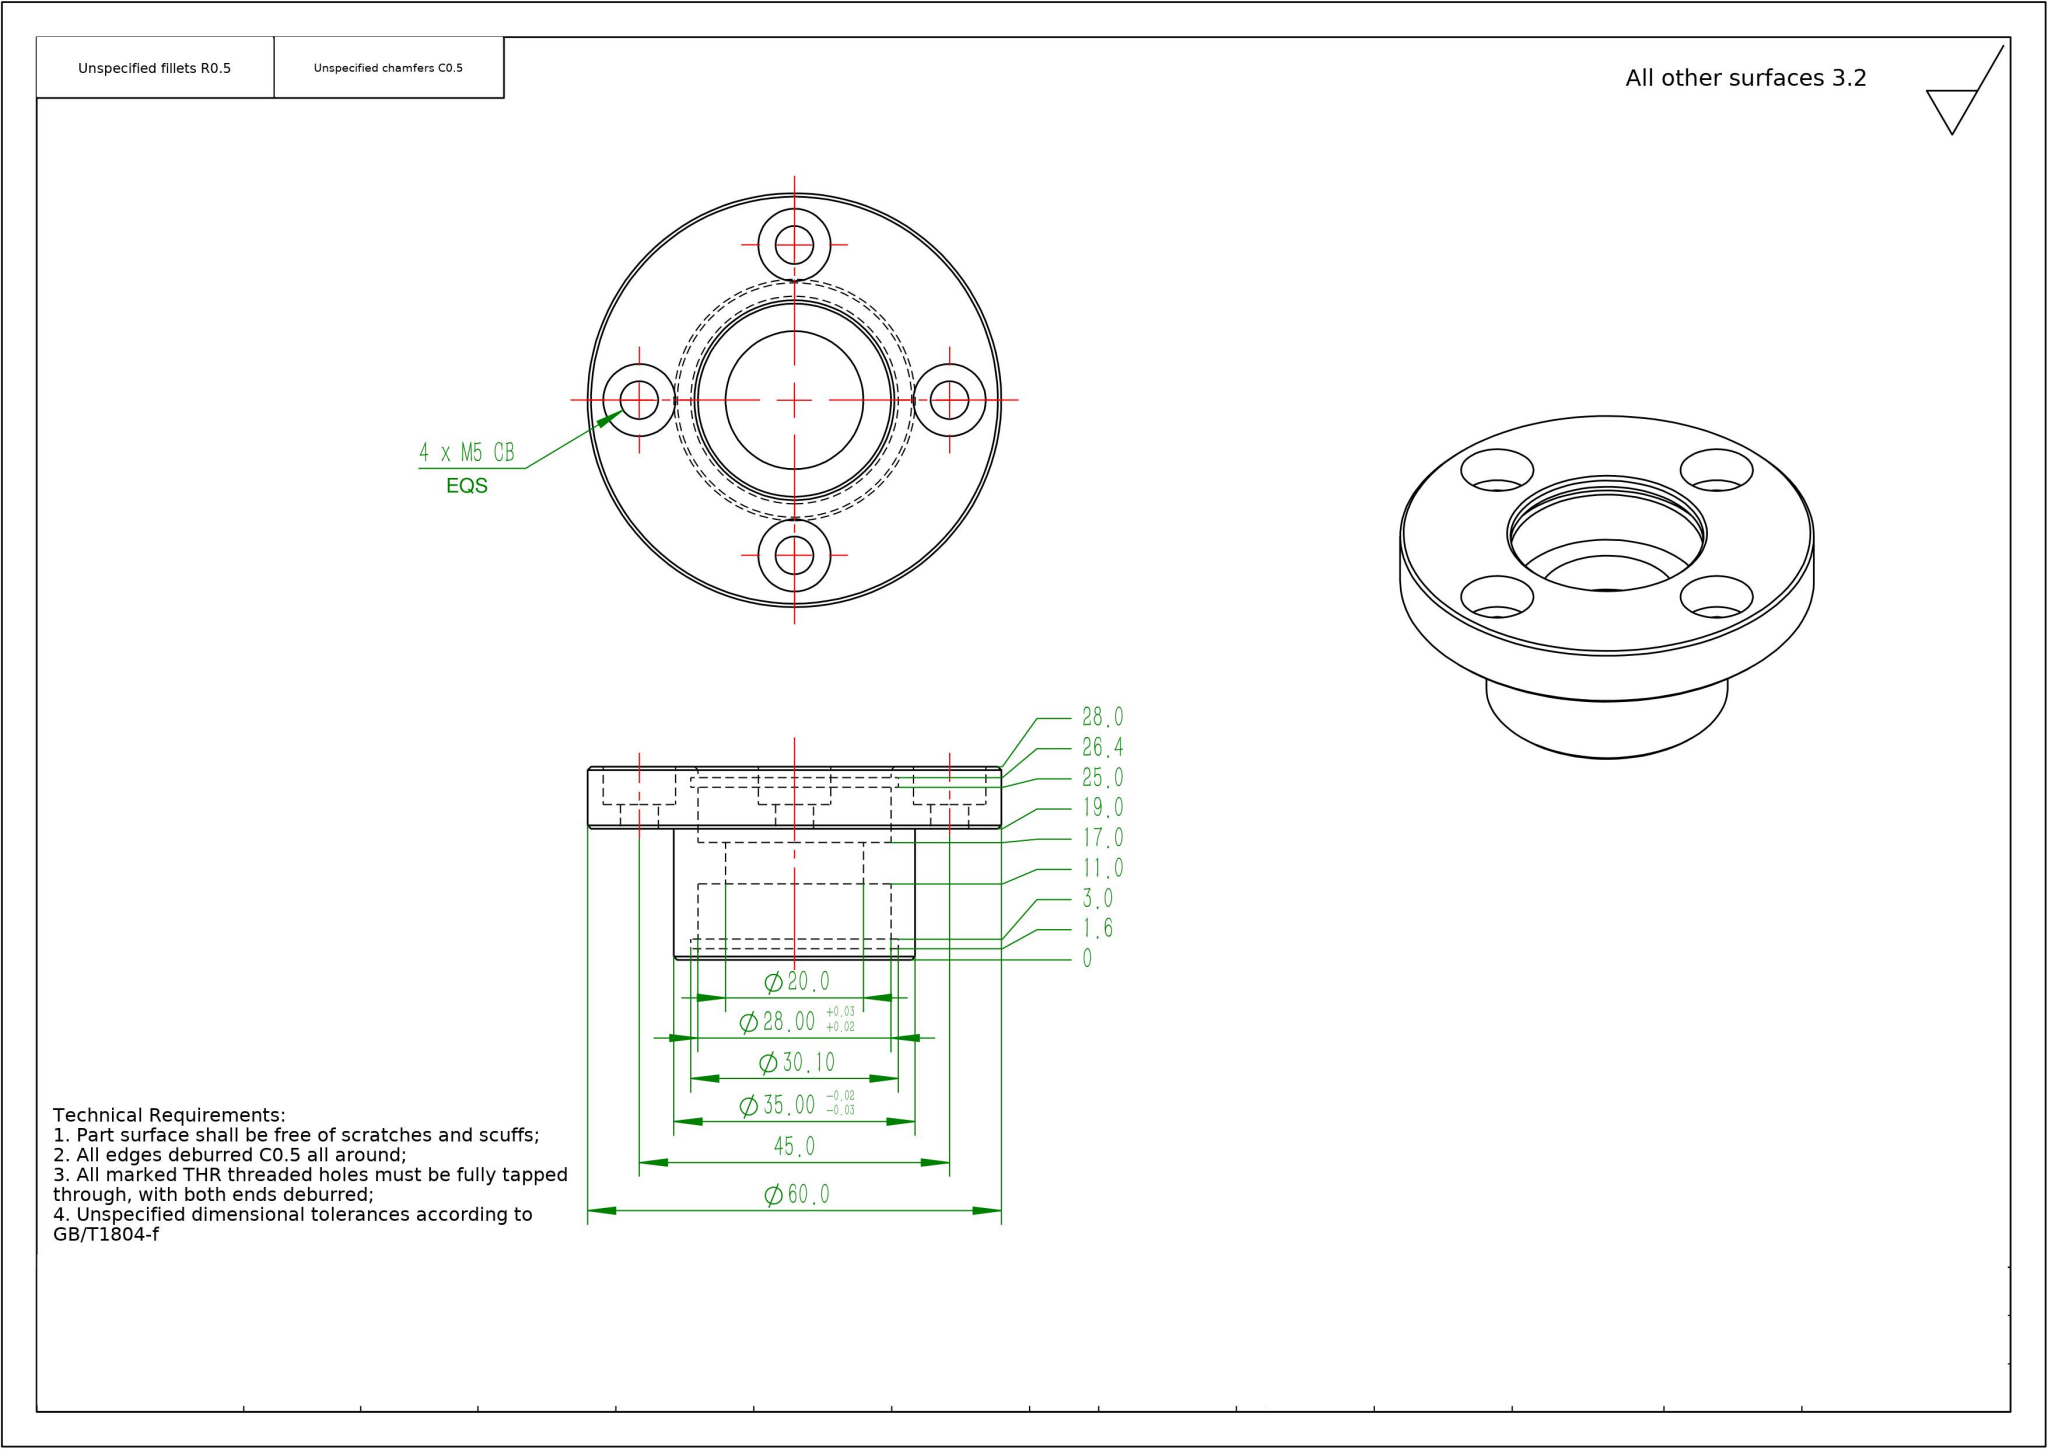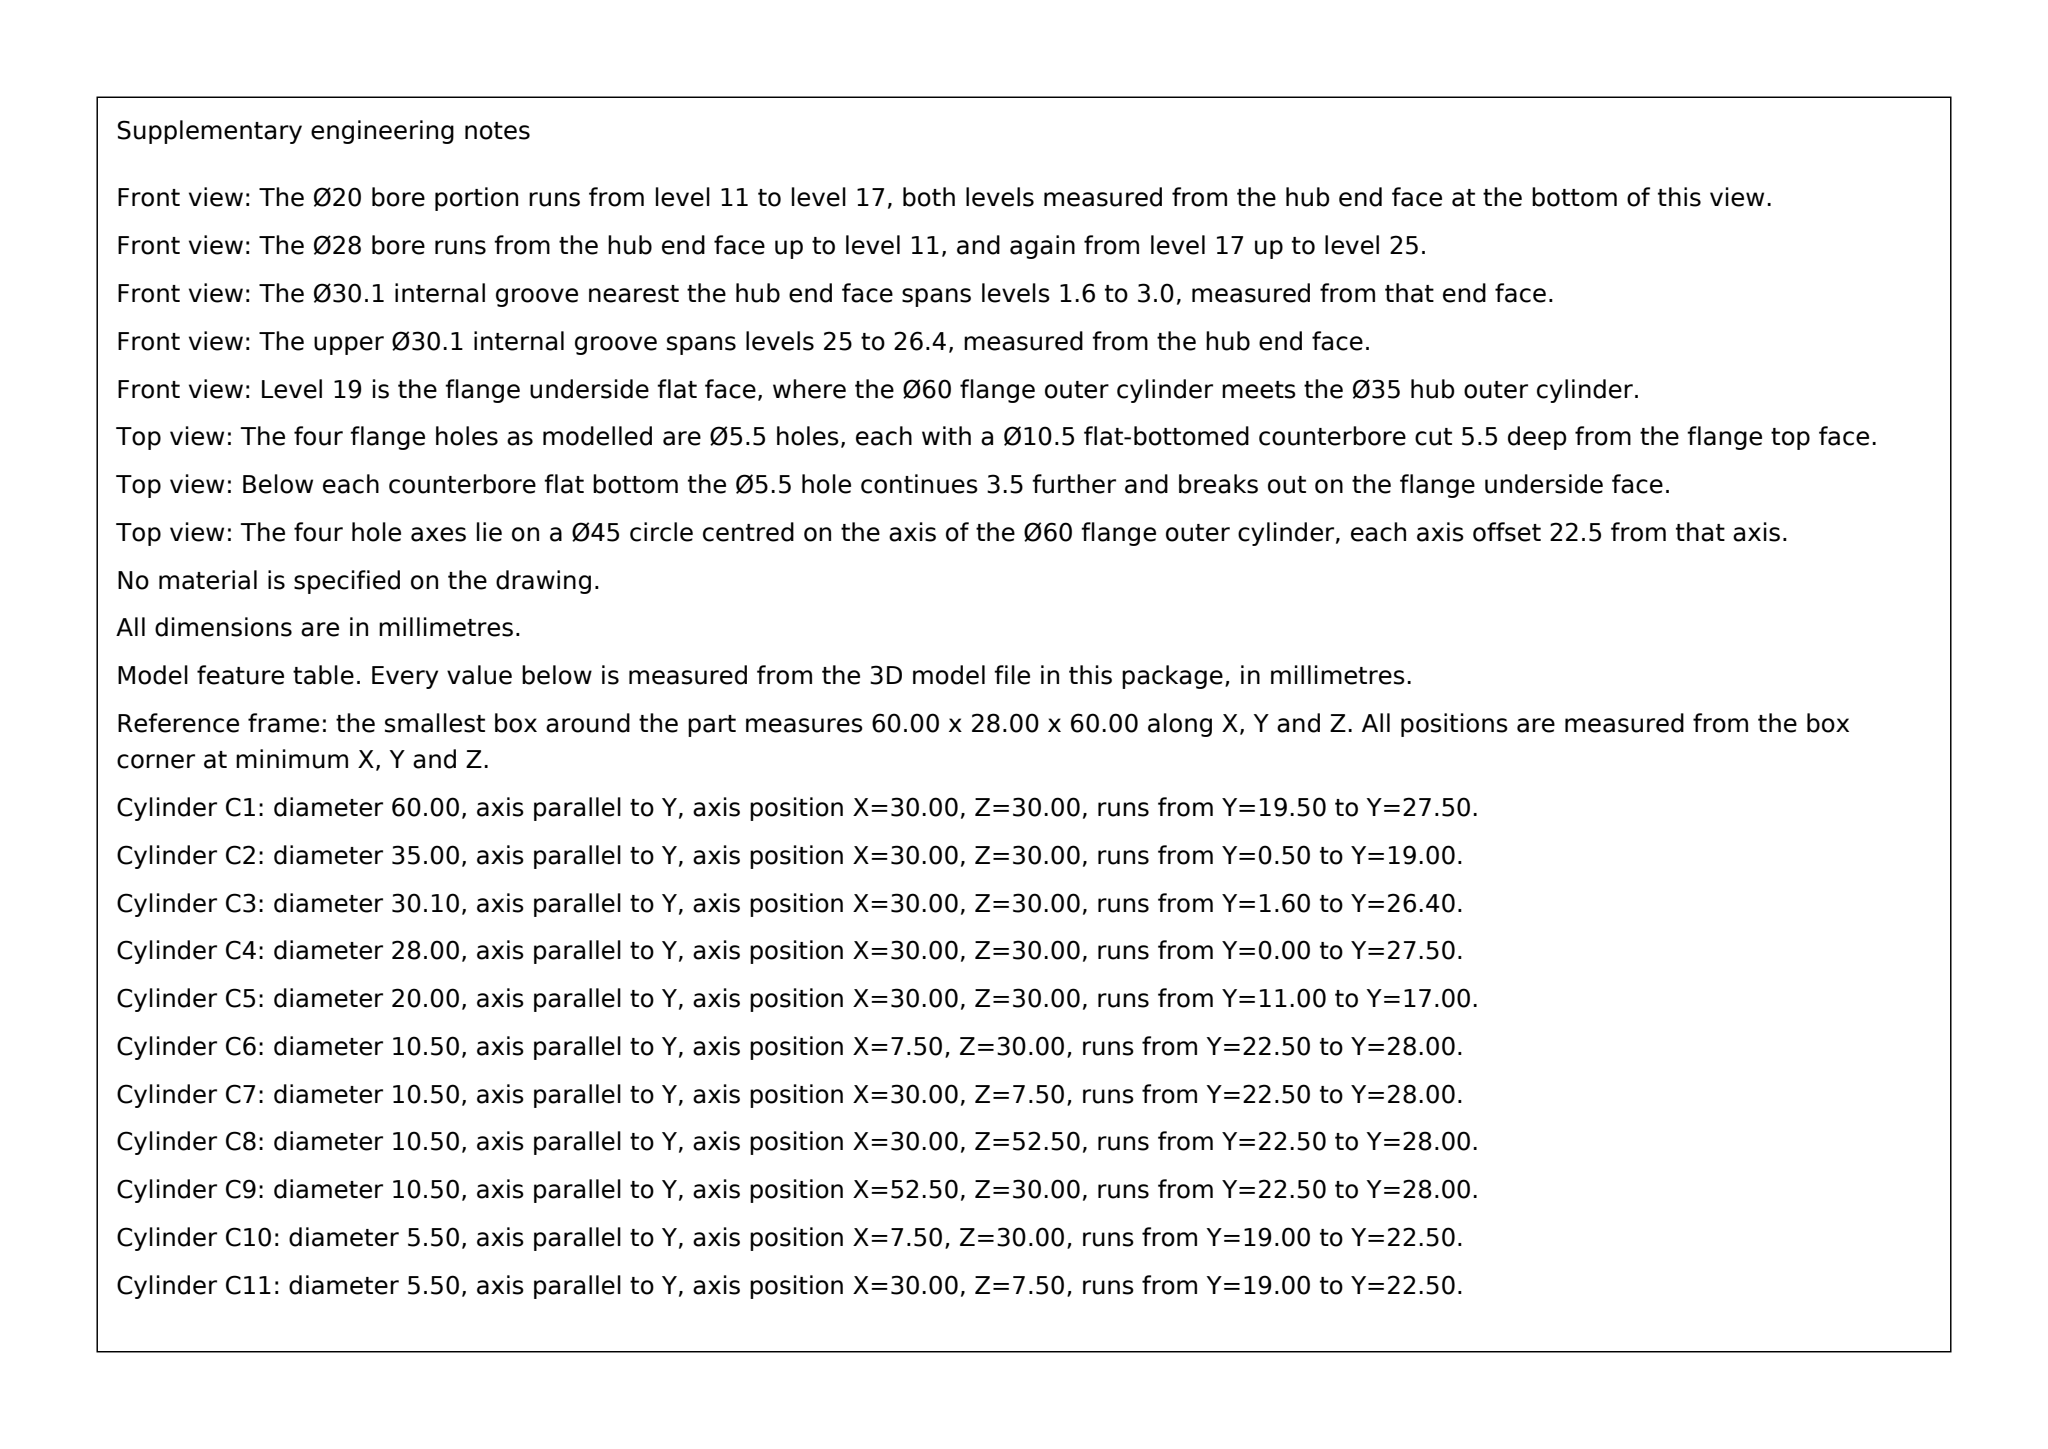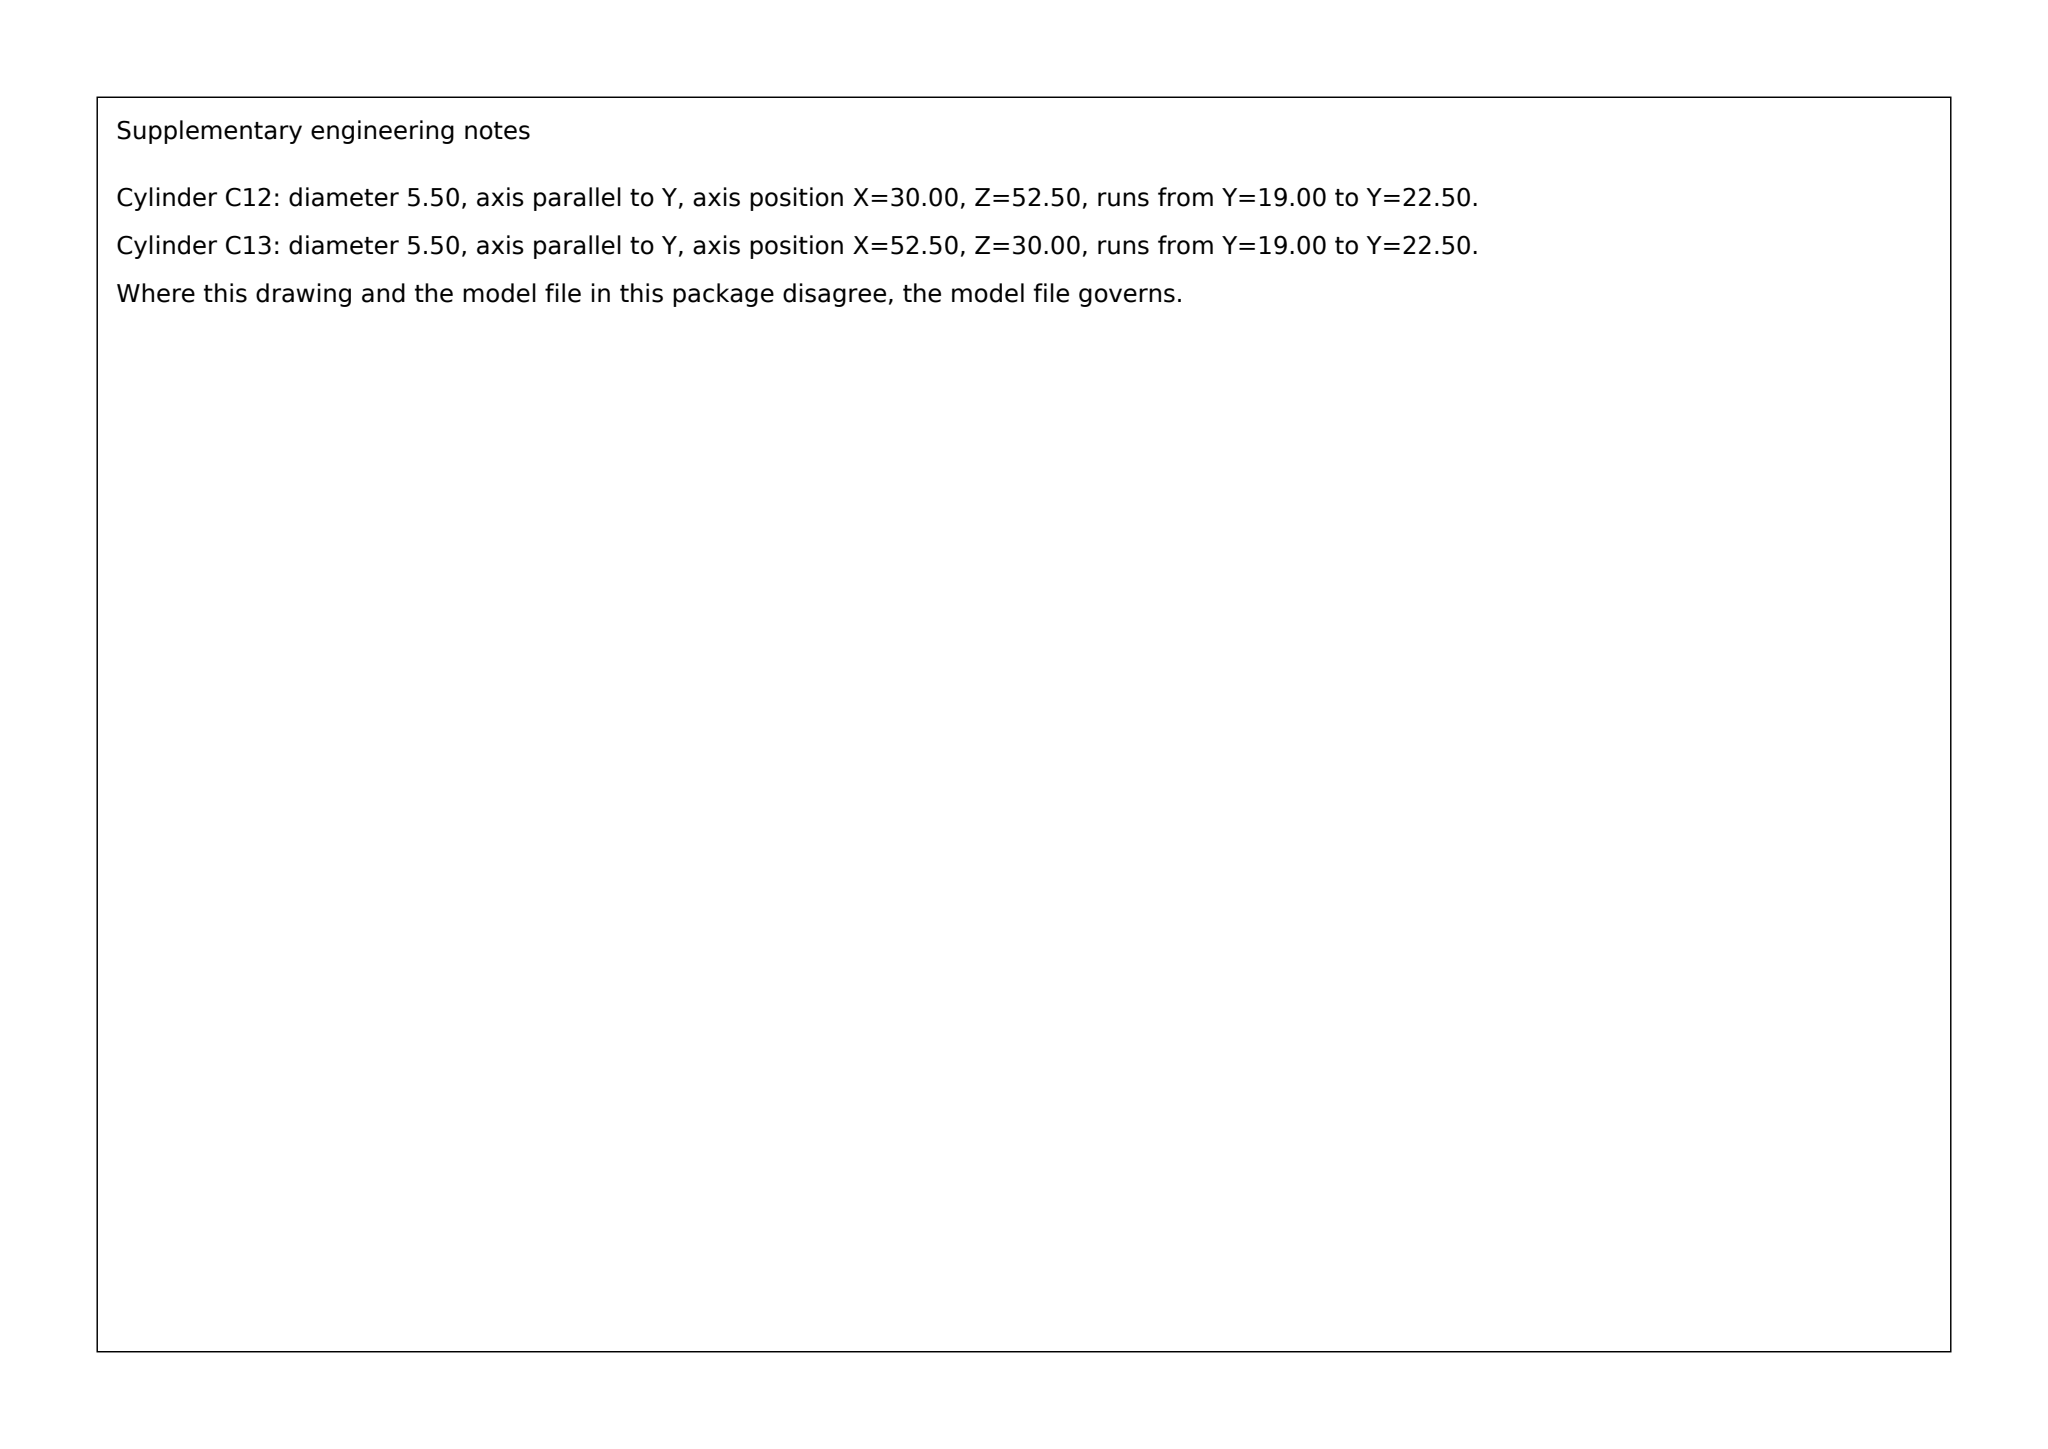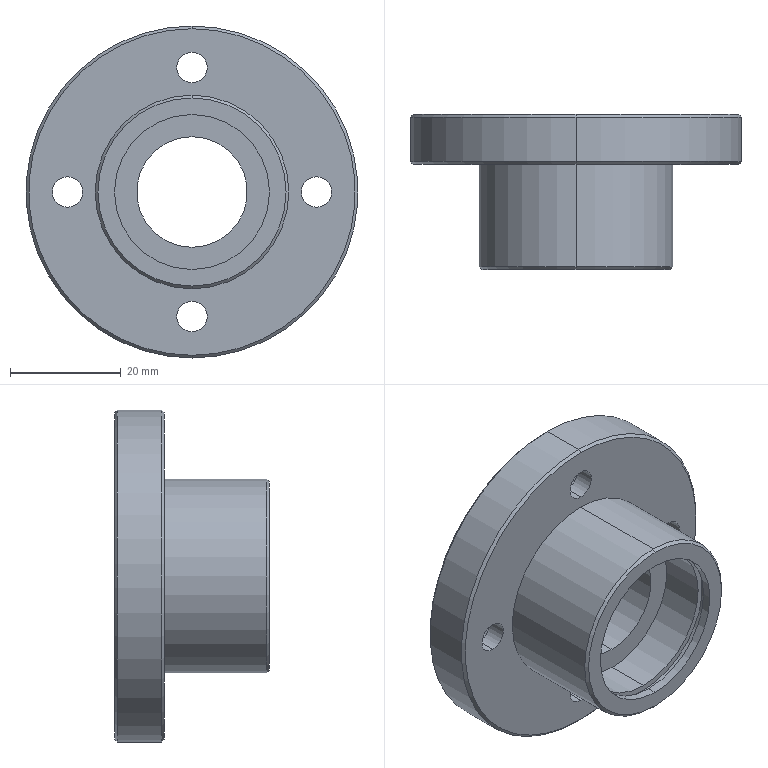Part | SolidWorks | mm | 1 solid | 55 faces | box 60 x 28 x 60 mm | volume 25718 mm3 | cylinder 34 | plane 13 | cone 8 | commonest cylinder face diameters 10.5 x8 28 x8 5.5 x8 30.1 x4 60 x2 20 x2 35 x2
Drawing notes:
4X C'BORE Ø10.5, EQ SP ON Ø45 B.C. | from the solid: cyl dia 10.5 axis y at (7.5,30),(30,7.5),(30,52.5),(52.5,30); R22.5 from axis (30,30) = Ø45 BC
4X C'BORE Ø10.5 DP 5.5 FROM 28.0 TOP FACE; FLOOR AT 22.5 | from the solid: cyl dia 10.5 len 5.5; planes y=28.0 (top) and y=22.5 (4X cbore floors)
4X Ø5.5 THRU TO C'BORE (22.5 TO 19.0 FLANGE UNDERSIDE) | from the solid: cyl dia 5.5 axis y len 3.5, between planes y=22.5 and y=19.0
INT THR MAJOR Ø30.10, THD LG 8.0 (17.0 TO 25.0 LEVELS) | from the solid: dia 30.10 thread-relief cyls (4) interleaved with dia 28.00 cyls len 8.0 between planes y=17.0 and y=25.0
INTERNAL THREAD: MAJOR Ø30.10, MINOR Ø28.00, FULL THD DP 8.0 | from the solid: Ø30.10 y-cyl L1.4 (thread crests) over Ø28.00 y-cyl L8.0, same axis at (30,30)
build123d program:
from build123d import *

# Parameters (mm, degrees)
SKETCH1_R           = 17.5
BOSS_EXTRUDE1_DEPTH = 28
SKETCH2_R           = 14
CUT_EXTRUDE1_DEPTH  = 11
SKETCH3_R           = 10
CUT_EXTRUDE2_DEPTH  = 31.025
CUT_EXTRUDE3_START  = -11
SKETCH4_R           = 14
CUT_EXTRUDE3_DEPTH  = 11
BOSS_EXTRUDE2_START = -9
SKETCH5_R           = 30
SKETCH5_R_2         = 17.5
BOSS_EXTRUDE2_DEPTH = 9
SKETCH6_R           = 2.75
CUT_EXTRUDE4_DEPTH  = 47.487
SKETCH7_R           = 5.25
CUT_EXTRUDE5_DEPTH  = 5.5
SKETCH8_R           = 15.05
CUT_EXTRUDE6_DEPTH  = 1.4
CUT_EXTRUDE7_START  = 1.4
SKETCH9_R           = 15.05
CUT_EXTRUDE7_DEPTH  = 1.4
CHAMFER1_SIZE       = 0.5


with BuildPart() as part:
    # Sketch1 → Boss-Extrude1 (new body)
    with BuildSketch(Plane(origin=(0, 0, 0), x_dir=(1, 0, 0), z_dir=(0, 1, 0))):
        with Locations(Location((0, 0, 0), (0, 0, 270))):
            Circle(SKETCH1_R)
    extrude(amount=BOSS_EXTRUDE1_DEPTH)

    # Sketch2 → Cut-Extrude1 (cut)
    with BuildSketch(Plane.XZ):
        with Locations(Location((0, 0, 0), (0, 0, 270))):
            Circle(SKETCH2_R)
    extrude(amount=-CUT_EXTRUDE1_DEPTH, mode=Mode.SUBTRACT)

    # Sketch3 → Cut-Extrude2 (cut, through all)
    with BuildSketch(Plane.XZ.offset(-11)):
        with Locations(Location((0, 0, 0), (0, 0, 270))):
            Circle(SKETCH3_R)
    extrude(amount=-CUT_EXTRUDE2_DEPTH, mode=Mode.SUBTRACT)

    # Sketch4 → Cut-Extrude3 (cut)
    with BuildSketch(Plane(origin=(0, 28, 0), x_dir=(1, 0, 0), z_dir=(0, 1, 0)).offset(CUT_EXTRUDE3_START)):
        with Locations(Location((0, 0, 0), (0, 0, 90))):
            Circle(SKETCH4_R)
    extrude(amount=CUT_EXTRUDE3_DEPTH, mode=Mode.SUBTRACT)

    # Sketch5 → Boss-Extrude2 (add)
    with BuildSketch(Plane(origin=(0, 28, 0), x_dir=(1, 0, 0), z_dir=(0, 1, 0)).offset(BOSS_EXTRUDE2_START)):
        with Locations(Location((0, 0, 0), (0, 0, 270))):
            Circle(SKETCH5_R)
        with Locations(Location((0, 0, 0), (0, 0, 270))):
            Circle(SKETCH5_R_2, mode=Mode.SUBTRACT)
    extrude(amount=BOSS_EXTRUDE2_DEPTH)

    # Sketch6 → Cut-Extrude4 (cut, through all)
    with BuildSketch(Plane.XZ.offset(-19)):
        with Locations(Location((0, 22.5, 0), (0, 0, 270))):
            Circle(SKETCH6_R)
        with Locations(Location((22.5, 0, 0), (0, 0, 270))):
            Circle(SKETCH6_R)
        with Locations(Location((-22.5, 0, 0), (0, 0, 270))):
            Circle(SKETCH6_R)
        with Locations(Location((0, -22.5, 0), (0, 0, 270))):
            Circle(SKETCH6_R)
    extrude(amount=-CUT_EXTRUDE4_DEPTH, mode=Mode.SUBTRACT)

    # Sketch7 → Cut-Extrude5 (cut)
    with BuildSketch(Plane(origin=(0, 28, 0), x_dir=(1, 0, 0), z_dir=(0, 1, 0))):
        with Locations(Location((-22.5, 0, 0), (0, 0, 270))):
            Circle(SKETCH7_R)
        with Locations(Location((0, 22.5, 0), (0, 0, 270))):
            Circle(SKETCH7_R)
        with Locations(Location((22.5, 0, 0), (0, 0, 270))):
            Circle(SKETCH7_R)
        with Locations(Location((0, -22.5, 0), (0, 0, 270))):
            Circle(SKETCH7_R)
    extrude(amount=-CUT_EXTRUDE5_DEPTH, mode=Mode.SUBTRACT)

    # Sketch8 → Cut-Extrude6 (cut)
    with BuildSketch(Plane(origin=(0, 3, 0), x_dir=(-1, 0, 0), z_dir=(0, -1, 0))):
        with Locations(Location((0, 0, 0), (0, 0, 90))):
            Circle(SKETCH8_R)
    extrude(amount=CUT_EXTRUDE6_DEPTH, mode=Mode.SUBTRACT)

    # Sketch9 → Cut-Extrude7 (cut)
    with BuildSketch(Plane(origin=(0, 25, 0), x_dir=(1, 0, 0), z_dir=(0, 1, 0)).offset(CUT_EXTRUDE7_START)):
        with Locations(Location((0, 0, 0), (0, 0, 90))):
            Circle(SKETCH9_R)
    extrude(amount=-CUT_EXTRUDE7_DEPTH, mode=Mode.SUBTRACT)

    # Chamfer1
    chamfer1_edges = [part.edges().sort_by_distance(p)[0] for p in [
        (0, 28, 14),
        (0, 0, -17.5),
        (0, 19, -30),
        (0, 28, -30),
    ]]
    chamfer(chamfer1_edges, length=CHAMFER1_SIZE)


solid = part.part